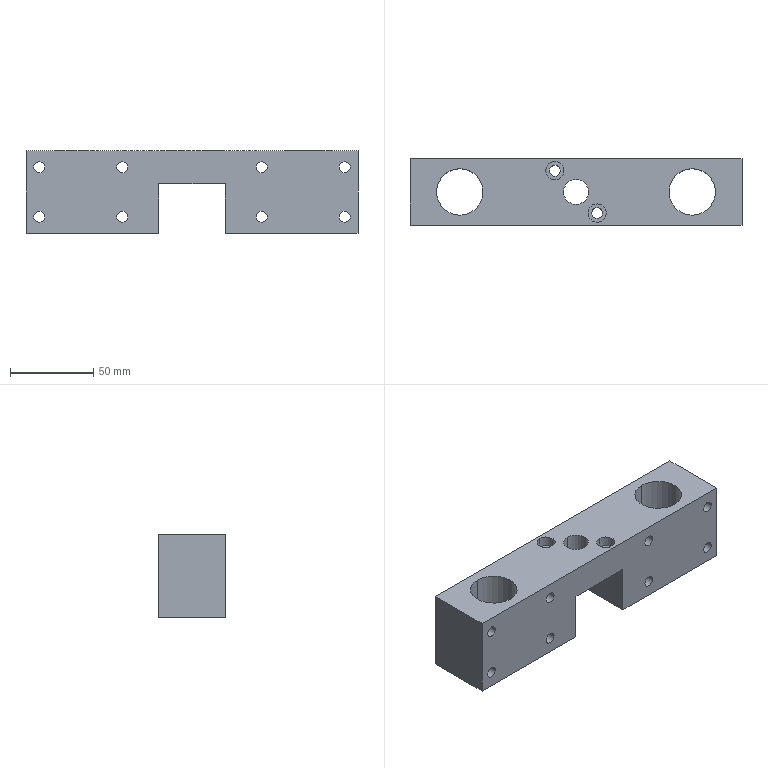Component | SolidWorks | YS01-056LiftingBearingHousing-ClampingAssembly-1 | 1 solid | 66 faces | box 200 x 40 x 49.8 mm | volume 269648 mm3 | cylinder 46 | plane 20 | commonest cylinder face diameters 11 x20 6.6 x20 28 x4 15 x2
build123d program:
from build123d import *

# Parameters (mm, degrees)
SKETCH1_W                                       = 200
SKETCH1_H                                       = 49.8
BOSS_EXTRUDE1_DEPTH                             = 40
SKETCH2_R                                       = 14
CUT_EXTRUDE1_DEPTH                              = 119.659
M6_HEX_SOCKET_HEAD_CAP_SCREW_CBORE1_D           = 6.6
M6_HEX_SOCKET_HEAD_CAP_SCREW_CBORE1_CBORE_D     = 11
M6_HEX_SOCKET_HEAD_CAP_SCREW_CBORE1_CBORE_DEPTH = 6.4
SKETCH6_R                                       = 7.5
CUT_EXTRUDE3_DEPTH                              = 119.659
SKETCH5_W                                       = 40
SKETCH5_H                                       = 59.6
CUT_EXTRUDE4_DEPTH                              = 146.28
M6_HEX_SOCKET_HEAD_CAP_SCREW_CBORE2_D           = 6.6
M6_HEX_SOCKET_HEAD_CAP_SCREW_CBORE2_CBORE_D     = 11
M6_HEX_SOCKET_HEAD_CAP_SCREW_CBORE2_CBORE_DEPTH = 6.4


with BuildPart() as part:
    # Sketch1 → Boss-Extrude1 (new body)
    with BuildSketch(Plane.XY):
        with Locations((0, 72.6)):
            Rectangle(SKETCH1_W, SKETCH1_H)
    extrude(amount=BOSS_EXTRUDE1_DEPTH)

    # Sketch2 → Cut-Extrude1 (cut, through all)
    with BuildSketch(Plane(origin=(0, 97.5, 0), x_dir=(1, 0, 0), z_dir=(0, 1, 0))):
        with Locations(Location((-70, -20, 0), (0, 0, 270))):
            Circle(SKETCH2_R)
        with Locations(Location((70, -20, 0), (0, 0, 270))):
            Circle(SKETCH2_R)
    extrude(amount=-CUT_EXTRUDE1_DEPTH, mode=Mode.SUBTRACT)

    # M6 Hex Socket Head Cap Screw CBORE1 (through all)
    with Locations(Plane.XY.offset(40)):
        with Locations((-92, 87.5), (-92, 57.7), (-42, 87.5), (-42, 57.7)):
            m6_hex_socket_head_cap_screw_cbore1 = CounterBoreHole(M6_HEX_SOCKET_HEAD_CAP_SCREW_CBORE1_D / 2, M6_HEX_SOCKET_HEAD_CAP_SCREW_CBORE1_CBORE_D / 2, M6_HEX_SOCKET_HEAD_CAP_SCREW_CBORE1_CBORE_DEPTH)

    # Mirror1: M6 Hex Socket Head Cap Screw CBORE1 across plane
    add(m6_hex_socket_head_cap_screw_cbore1.mirror(Plane.ZY), mode=Mode.SUBTRACT)

    # Sketch6 → Cut-Extrude3 (cut, through all)
    with BuildSketch(Plane(origin=(0, 97.5, 0), x_dir=(1, 0, 0), z_dir=(0, 1, 0))):
        with Locations(Location((0, -20, 0), (0, 0, 270))):
            Circle(SKETCH6_R)
    extrude(amount=-CUT_EXTRUDE3_DEPTH, mode=Mode.SUBTRACT)

    # Sketch5 → Cut-Extrude4 (cut, through all)
    with BuildSketch(Plane.XY.offset(40)):
        with Locations((0, 47.7)):
            Rectangle(SKETCH5_W, SKETCH5_H)
    extrude(amount=-CUT_EXTRUDE4_DEPTH, mode=Mode.SUBTRACT)

    # M6 Hex Socket Head Cap Screw CBORE2 (through all)
    with Locations(Plane(origin=(0, 97.5, 0), x_dir=(1, 0, 0), z_dir=(0, 1, 0))):
        with Locations((-12.728, -7.272), (12.728, -32.728)):
            CounterBoreHole(M6_HEX_SOCKET_HEAD_CAP_SCREW_CBORE2_D / 2, M6_HEX_SOCKET_HEAD_CAP_SCREW_CBORE2_CBORE_D / 2, M6_HEX_SOCKET_HEAD_CAP_SCREW_CBORE2_CBORE_DEPTH)


solid = part.part

# Placed as in the assembly
solid = solid.moved(Location((-566.612, -143.873, 2388.4), (-90, 0, 180)))